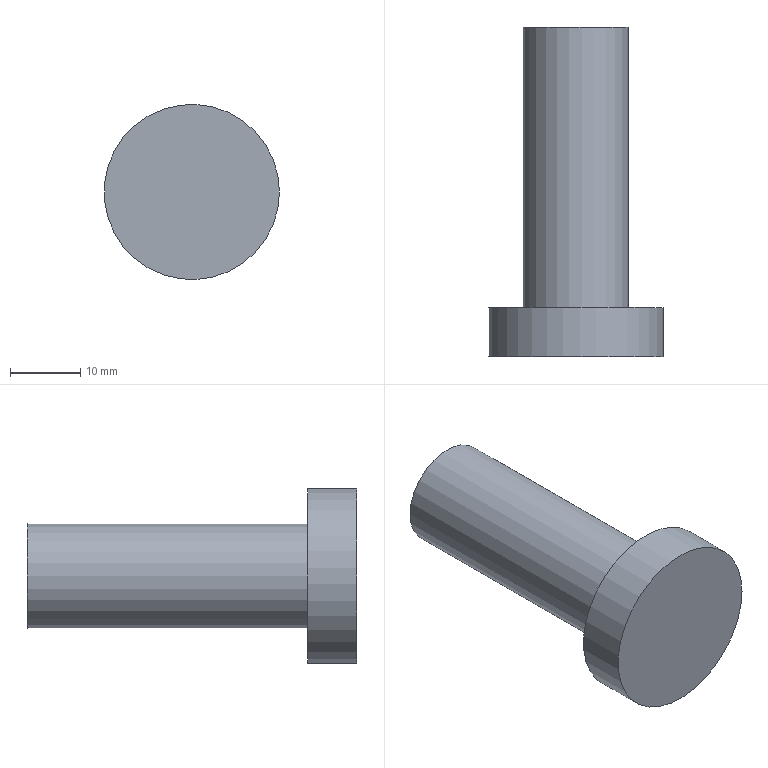Component | NX | BOLT | 1 solid | 5 faces | box 25 x 47 x 25 mm | volume 10505 mm3 | plane 3 | cylinder 2 | commonest cylinder face diameters 15 x1 25 x1
STEP:
#1=CARTESIAN_POINT('',(0.,0.,0.));
#2=DIRECTION('',(0.,0.,1.));
#3=DIRECTION('',(1.,0.,0.));
#4=AXIS2_PLACEMENT_3D('',#1,#2,#3);
#5=CARTESIAN_POINT('',(113.364,37.126,980.));
#6=VERTEX_POINT('',#5);
#7=CARTESIAN_POINT('',(105.864,37.126,980.));
#8=DIRECTION('',(0.,-1.,0.));
#9=DIRECTION('',(1.,0.,0.));
#10=AXIS2_PLACEMENT_3D('',#7,#8,#9);
#11=CIRCLE('',#10,7.5);
#12=CARTESIAN_POINT('',(105.864,37.126,980.));
#13=DIRECTION('',(0.,1.,0.));
#14=DIRECTION('',(-1.,0.,0.));
#15=AXIS2_PLACEMENT_3D('',#12,#13,#14);
#16=PLANE('',#15);
#17=CARTESIAN_POINT('',(-7.5,0.));
#18=CARTESIAN_POINT('',(-7.5,12.99));
#19=CARTESIAN_POINT('',(3.75,6.495));
#20=CARTESIAN_POINT('',(15.,0.));
#21=CARTESIAN_POINT('',(3.75,-6.495));
#22=CARTESIAN_POINT('',(-7.5,-12.99));
#23=CARTESIAN_POINT('',(-7.5,0.));
#24=(BOUNDED_CURVE()B_SPLINE_CURVE(2,(#17,#18,#19,#20,#21,#22,#23),.UNSPECIFIED.,.T.,.F.)B_SPLINE_CURVE_WITH_KNOTS((1,2,2,2,2,1),(-2.094,0.,2.094,4.189,6.283,8.378),.UNSPECIFIED.)CURVE()GEOMETRIC_REPRESENTATION_ITEM()RATIONAL_B_SPLINE_CURVE((1.,0.5,1.,0.5,1.,0.5,1.))REPRESENTATION_ITEM(''));
#25=(GEOMETRIC_REPRESENTATION_CONTEXT(2)PARAMETRIC_REPRESENTATION_CONTEXT()REPRESENTATION_CONTEXT('',''));
#26=DEFINITIONAL_REPRESENTATION('',(#24),#25);
#27=PCURVE('',#16,#26);
#28=CARTESIAN_POINT('',(105.864,37.126,980.));
#29=DIRECTION('',(0.,-1.,0.));
#30=DIRECTION('',(1.,0.,0.));
#31=AXIS2_PLACEMENT_3D('',#28,#29,#30);
#32=CYLINDRICAL_SURFACE('',#31,7.5);
#33=CARTESIAN_POINT('',(0.,0.));
#34=DIRECTION('',(1.,0.));
#35=VECTOR('',#34,1.);
#36=LINE('',#33,#35);
#37=(GEOMETRIC_REPRESENTATION_CONTEXT(2)PARAMETRIC_REPRESENTATION_CONTEXT()REPRESENTATION_CONTEXT('',''));
#38=DEFINITIONAL_REPRESENTATION('',(#36),#37);
#39=PCURVE('',#32,#38);
#40=SURFACE_CURVE('',#11,(#27,#39),.PCURVE_S1.);
#41=EDGE_CURVE('',#6,#6,#40,.T.);
#42=ORIENTED_EDGE('',*,*,#41,.F.);
#43=EDGE_LOOP('',(#42));
#44=FACE_BOUND('',#43,.T.);
#45=ADVANCED_FACE('',(#44),#16,.T.);
#46=CARTESIAN_POINT('',(113.364,-2.874,980.));
#47=VERTEX_POINT('',#46);
#48=CARTESIAN_POINT('',(105.864,-2.874,980.));
#49=DIRECTION('',(0.,1.,0.));
#50=DIRECTION('',(1.,0.,0.));
#51=AXIS2_PLACEMENT_3D('',#48,#49,#50);
#52=CIRCLE('',#51,7.5);
#53=CARTESIAN_POINT('',(6.283,40.));
#54=DIRECTION('',(-1.,0.));
#55=VECTOR('',#54,1.);
#56=LINE('',#53,#55);
#57=(GEOMETRIC_REPRESENTATION_CONTEXT(2)PARAMETRIC_REPRESENTATION_CONTEXT()REPRESENTATION_CONTEXT('',''));
#58=DEFINITIONAL_REPRESENTATION('',(#56),#57);
#59=PCURVE('',#32,#58);
#60=CARTESIAN_POINT('',(105.864,-2.874,980.));
#61=DIRECTION('',(0.,-1.,0.));
#62=DIRECTION('',(1.,0.,0.));
#63=AXIS2_PLACEMENT_3D('',#60,#61,#62);
#64=PLANE('',#63);
#65=CARTESIAN_POINT('',(7.5,0.));
#66=CARTESIAN_POINT('',(7.5,-12.99));
#67=CARTESIAN_POINT('',(-3.75,-6.495));
#68=CARTESIAN_POINT('',(-15.,-0.));
#69=CARTESIAN_POINT('',(-3.75,6.495));
#70=CARTESIAN_POINT('',(7.5,12.99));
#71=CARTESIAN_POINT('',(7.5,0.));
#72=(BOUNDED_CURVE()B_SPLINE_CURVE(2,(#65,#66,#67,#68,#69,#70,#71),.UNSPECIFIED.,.T.,.F.)B_SPLINE_CURVE_WITH_KNOTS((1,2,2,2,2,1),(-2.094,0.,2.094,4.189,6.283,8.378),.UNSPECIFIED.)CURVE()GEOMETRIC_REPRESENTATION_ITEM()RATIONAL_B_SPLINE_CURVE((1.,0.5,1.,0.5,1.,0.5,1.))REPRESENTATION_ITEM(''));
#73=(GEOMETRIC_REPRESENTATION_CONTEXT(2)PARAMETRIC_REPRESENTATION_CONTEXT()REPRESENTATION_CONTEXT('',''));
#74=DEFINITIONAL_REPRESENTATION('',(#72),#73);
#75=PCURVE('',#64,#74);
#76=SURFACE_CURVE('',#52,(#59,#75),.PCURVE_S1.);
#77=EDGE_CURVE('',#47,#47,#76,.T.);
#78=ORIENTED_EDGE('',*,*,#77,.T.);
#79=CARTESIAN_POINT('',(113.364,37.126,980.));
#80=CARTESIAN_POINT('',(113.364,-2.874,980.));
#81=B_SPLINE_CURVE_WITH_KNOTS('',1,(#79,#80),.UNSPECIFIED.,.F.,.F.,(2,2),(0.,40.),.PIECEWISE_BEZIER_KNOTS.);
#82=CARTESIAN_POINT('',(0.,0.));
#83=DIRECTION('',(0.,1.));
#84=VECTOR('',#83,1.);
#85=LINE('',#82,#84);
#86=(GEOMETRIC_REPRESENTATION_CONTEXT(2)PARAMETRIC_REPRESENTATION_CONTEXT()REPRESENTATION_CONTEXT('',''));
#87=DEFINITIONAL_REPRESENTATION('',(#85),#86);
#88=PCURVE('',#32,#87);
#89=CARTESIAN_POINT('',(6.283,0.));
#90=DIRECTION('',(0.,1.));
#91=VECTOR('',#90,1.);
#92=LINE('',#89,#91);
#93=(GEOMETRIC_REPRESENTATION_CONTEXT(2)PARAMETRIC_REPRESENTATION_CONTEXT()REPRESENTATION_CONTEXT('',''));
#94=DEFINITIONAL_REPRESENTATION('',(#92),#93);
#95=PCURVE('',#32,#94);
#96=SEAM_CURVE('',#81,(#88,#95),.PCURVE_S1.);
#97=EDGE_CURVE('',#6,#47,#96,.T.);
#98=ORIENTED_EDGE('',*,*,#97,.F.);
#99=ORIENTED_EDGE('',*,*,#41,.T.);
#100=ORIENTED_EDGE('',*,*,#97,.T.);
#101=EDGE_LOOP('',(#78,#98,#99,#100));
#102=FACE_BOUND('',#101,.T.);
#103=ADVANCED_FACE('',(#102),#32,.T.);
#104=CARTESIAN_POINT('',(118.364,-9.874,980.));
#105=VERTEX_POINT('',#104);
#106=CARTESIAN_POINT('',(105.864,-9.874,980.));
#107=DIRECTION('',(0.,-1.,0.));
#108=DIRECTION('',(1.,0.,0.));
#109=AXIS2_PLACEMENT_3D('',#106,#107,#108);
#110=CIRCLE('',#109,12.5);
#111=CARTESIAN_POINT('',(105.864,-9.874,980.));
#112=DIRECTION('',(0.,1.,0.));
#113=DIRECTION('',(-1.,0.,0.));
#114=AXIS2_PLACEMENT_3D('',#111,#112,#113);
#115=CYLINDRICAL_SURFACE('',#114,12.5);
#116=CARTESIAN_POINT('',(9.425,0.));
#117=DIRECTION('',(-1.,0.));
#118=VECTOR('',#117,1.);
#119=LINE('',#116,#118);
#120=(GEOMETRIC_REPRESENTATION_CONTEXT(2)PARAMETRIC_REPRESENTATION_CONTEXT()REPRESENTATION_CONTEXT('',''));
#121=DEFINITIONAL_REPRESENTATION('',(#119),#120);
#122=PCURVE('',#115,#121);
#123=CARTESIAN_POINT('',(105.864,-9.874,980.));
#124=DIRECTION('',(0.,-1.,0.));
#125=DIRECTION('',(1.,0.,0.));
#126=AXIS2_PLACEMENT_3D('',#123,#124,#125);
#127=PLANE('',#126);
#128=CARTESIAN_POINT('',(0.,0.));
#129=DIRECTION('',(1.,0.));
#130=AXIS2_PLACEMENT_2D('',#128,#129);
#131=CIRCLE('',#130,12.5);
#132=(GEOMETRIC_REPRESENTATION_CONTEXT(2)PARAMETRIC_REPRESENTATION_CONTEXT()REPRESENTATION_CONTEXT('',''));
#133=DEFINITIONAL_REPRESENTATION('',(#131),#132);
#134=PCURVE('',#127,#133);
#135=SURFACE_CURVE('',#110,(#122,#134),.PCURVE_S1.);
#136=EDGE_CURVE('',#105,#105,#135,.T.);
#137=ORIENTED_EDGE('',*,*,#136,.F.);
#138=CARTESIAN_POINT('',(118.364,-2.874,980.));
#139=VERTEX_POINT('',#138);
#140=CARTESIAN_POINT('',(118.364,-9.874,980.));
#141=CARTESIAN_POINT('',(118.364,-2.874,980.));
#142=B_SPLINE_CURVE_WITH_KNOTS('',1,(#140,#141),.UNSPECIFIED.,.F.,.F.,(2,2),(0.,7.),.PIECEWISE_BEZIER_KNOTS.);
#143=CARTESIAN_POINT('',(9.425,0.));
#144=DIRECTION('',(0.,1.));
#145=VECTOR('',#144,1.);
#146=LINE('',#143,#145);
#147=(GEOMETRIC_REPRESENTATION_CONTEXT(2)PARAMETRIC_REPRESENTATION_CONTEXT()REPRESENTATION_CONTEXT('',''));
#148=DEFINITIONAL_REPRESENTATION('',(#146),#147);
#149=PCURVE('',#115,#148);
#150=CARTESIAN_POINT('',(3.142,0.));
#151=DIRECTION('',(0.,1.));
#152=VECTOR('',#151,1.);
#153=LINE('',#150,#152);
#154=(GEOMETRIC_REPRESENTATION_CONTEXT(2)PARAMETRIC_REPRESENTATION_CONTEXT()REPRESENTATION_CONTEXT('',''));
#155=DEFINITIONAL_REPRESENTATION('',(#153),#154);
#156=PCURVE('',#115,#155);
#157=SEAM_CURVE('',#142,(#149,#156),.PCURVE_S1.);
#158=EDGE_CURVE('',#105,#139,#157,.T.);
#159=ORIENTED_EDGE('',*,*,#158,.T.);
#160=CARTESIAN_POINT('',(105.864,-2.874,980.));
#161=DIRECTION('',(0.,-1.,0.));
#162=DIRECTION('',(1.,0.,0.));
#163=AXIS2_PLACEMENT_3D('',#160,#161,#162);
#164=CIRCLE('',#163,12.5);
#165=CARTESIAN_POINT('',(9.425,7.));
#166=DIRECTION('',(-1.,0.));
#167=VECTOR('',#166,1.);
#168=LINE('',#165,#167);
#169=(GEOMETRIC_REPRESENTATION_CONTEXT(2)PARAMETRIC_REPRESENTATION_CONTEXT()REPRESENTATION_CONTEXT('',''));
#170=DEFINITIONAL_REPRESENTATION('',(#168),#169);
#171=PCURVE('',#115,#170);
#172=CARTESIAN_POINT('',(0.,0.));
#173=DIRECTION('',(1.,0.));
#174=AXIS2_PLACEMENT_2D('',#172,#173);
#175=CIRCLE('',#174,12.5);
#176=(GEOMETRIC_REPRESENTATION_CONTEXT(2)PARAMETRIC_REPRESENTATION_CONTEXT()REPRESENTATION_CONTEXT('',''));
#177=DEFINITIONAL_REPRESENTATION('',(#175),#176);
#178=PCURVE('',#64,#177);
#179=SURFACE_CURVE('',#164,(#171,#178),.PCURVE_S1.);
#180=EDGE_CURVE('',#139,#139,#179,.T.);
#181=ORIENTED_EDGE('',*,*,#180,.T.);
#182=ORIENTED_EDGE('',*,*,#158,.F.);
#183=EDGE_LOOP('',(#137,#159,#181,#182));
#184=FACE_BOUND('',#183,.T.);
#185=ADVANCED_FACE('',(#184),#115,.T.);
#186=ORIENTED_EDGE('',*,*,#136,.T.);
#187=EDGE_LOOP('',(#186));
#188=FACE_BOUND('',#187,.T.);
#189=ADVANCED_FACE('',(#188),#127,.T.);
#190=ORIENTED_EDGE('',*,*,#77,.F.);
#191=EDGE_LOOP('',(#190));
#192=FACE_BOUND('',#191,.T.);
#193=ORIENTED_EDGE('',*,*,#180,.F.);
#194=EDGE_LOOP('',(#193));
#195=FACE_BOUND('',#194,.T.);
#196=ADVANCED_FACE('',(#192,#195),#64,.F.);
#197=CLOSED_SHELL('',(#45,#103,#185,#189,#196));
#198=MANIFOLD_SOLID_BREP('',#197);
#199=(LENGTH_UNIT()NAMED_UNIT(*)SI_UNIT(.MILLI.,.METRE.));
#200=UNCERTAINTY_MEASURE_WITH_UNIT(LENGTH_MEASURE(0.00001),#199,'','');
#201=(NAMED_UNIT(*)PLANE_ANGLE_UNIT()SI_UNIT($,.RADIAN.));
#202=(NAMED_UNIT(*)SI_UNIT($,.STERADIAN.)SOLID_ANGLE_UNIT());
#203=(GEOMETRIC_REPRESENTATION_CONTEXT(3)GLOBAL_UNCERTAINTY_ASSIGNED_CONTEXT((#200))GLOBAL_UNIT_ASSIGNED_CONTEXT((#199,#201,#202))REPRESENTATION_CONTEXT('',''));
#204=ADVANCED_BREP_SHAPE_REPRESENTATION('',(#4,#198),#203);